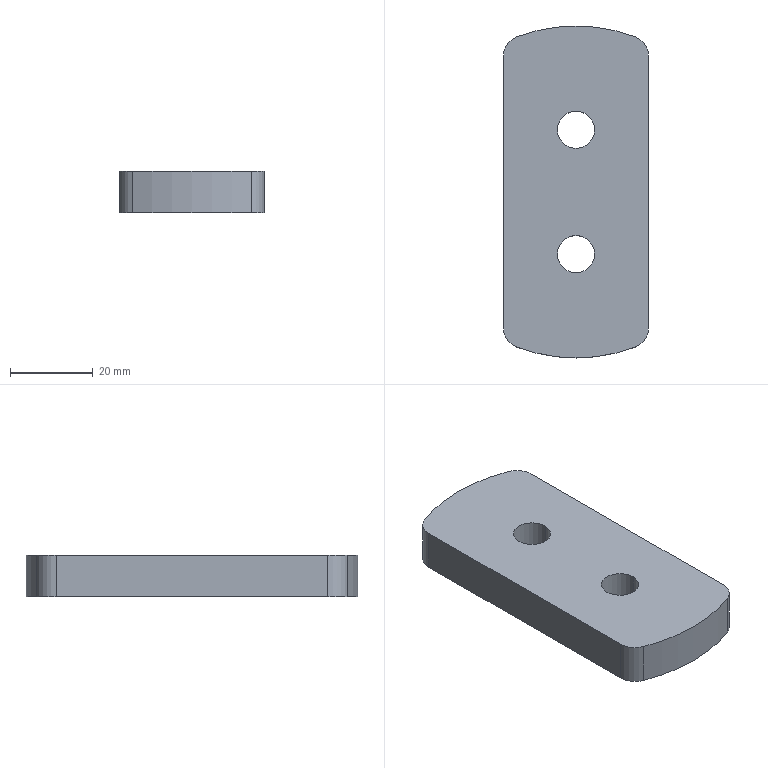Component | SolidWorks | NewTypeCurveBenderReinforcementWheelStopCover-DoubleWheel-1 | 1 solid | 14 faces | box 35 x 80 x 10 mm | volume 25728 mm3 | cylinder 10 | plane 4 | commonest cylinder face diameters 9 x4 10 x4 80 x2
build123d program:
from build123d import *

# Parameters (mm, degrees)
SKETCH1_R           = 4.5
BOSS_EXTRUDE1_DEPTH = 10


with BuildPart() as part:
    # Sketch1 → Boss-Extrude1 (new body)
    with BuildSketch(Plane.XY):
        with BuildLine():
            Line((-17.5, 32.692), (-17.5, -32.692))
            ThreePointArc((-17.5, -32.692), (-16.619, -35.526), (-14.286, -37.362))
            ThreePointArc((-14.286, -37.362), (0, -40), (14.286, -37.362))
            ThreePointArc((14.286, -37.362), (16.619, -35.526), (17.5, -32.692))
            Line((17.5, -32.692), (17.5, 32.692))
            ThreePointArc((17.5, 32.692), (16.619, 35.526), (14.286, 37.362))
            ThreePointArc((14.286, 37.362), (0, 40), (-14.286, 37.362))
            ThreePointArc((-14.286, 37.362), (-16.619, 35.526), (-17.5, 32.692))
        make_face()
        with Locations((0, 15)):
            Circle(SKETCH1_R, mode=Mode.SUBTRACT)
        with Locations(Location((0, -15, 0), (0, 0, 180))):
            Circle(SKETCH1_R, mode=Mode.SUBTRACT)
    extrude(amount=BOSS_EXTRUDE1_DEPTH)


solid = part.part

# Placed as in the assembly
solid = solid.moved(Location((50, -204, 59), (0, 0, 0)))
STEP:
#1=COLOUR_RGB('',0.7922,0.8196,0.9333);
#2=FILL_AREA_STYLE_COLOUR('',#1);
#3=FILL_AREA_STYLE('',(#2));
#4=SURFACE_STYLE_FILL_AREA(#3);
#5=SURFACE_SIDE_STYLE('',(#4));
#6=SURFACE_STYLE_USAGE(.BOTH.,#5);
#7=PRESENTATION_STYLE_ASSIGNMENT((#6));
#8=CARTESIAN_POINT('',(2.146,-8.622,2.323));
#9=VERTEX_POINT('',#8);
#10=CARTESIAN_POINT('',(1.791,-8.622,2.323));
#11=VERTEX_POINT('',#10);
#12=CARTESIAN_POINT('',(1.969,-8.622,2.323));
#13=DIRECTION('',(-0.,0.,-1.));
#14=DIRECTION('',(1.,0.,-0.));
#15=AXIS2_PLACEMENT_3D('',#12,#13,#14);
#16=CIRCLE('',#15,0.1772);
#17=EDGE_CURVE('',#9,#11,#16,.T.);
#18=ORIENTED_EDGE('',*,*,#17,.T.);
#19=CARTESIAN_POINT('',(1.791,-8.622,2.717));
#20=VERTEX_POINT('',#19);
#21=CARTESIAN_POINT('',(1.791,-8.622,2.323));
#22=DIRECTION('',(0.,-0.,1.));
#23=VECTOR('',#22,39.37);
#24=LINE('',#21,#23);
#25=EDGE_CURVE('',#11,#20,#24,.T.);
#26=ORIENTED_EDGE('',*,*,#25,.T.);
#27=CARTESIAN_POINT('',(2.146,-8.622,2.717));
#28=VERTEX_POINT('',#27);
#29=CARTESIAN_POINT('',(1.969,-8.622,2.717));
#30=DIRECTION('',(-0.,0.,-1.));
#31=DIRECTION('',(1.,0.,-0.));
#32=AXIS2_PLACEMENT_3D('',#29,#30,#31);
#33=CIRCLE('',#32,0.1772);
#34=EDGE_CURVE('',#28,#20,#33,.T.);
#35=ORIENTED_EDGE('',*,*,#34,.F.);
#36=CARTESIAN_POINT('',(2.146,-8.622,2.323));
#37=DIRECTION('',(0.,-0.,1.));
#38=VECTOR('',#37,39.37);
#39=LINE('',#36,#38);
#40=EDGE_CURVE('',#9,#28,#39,.T.);
#41=ORIENTED_EDGE('',*,*,#40,.F.);
#42=EDGE_LOOP('',(#18,#26,#35,#41));
#43=FACE_OUTER_BOUND('',#42,.T.);
#44=CARTESIAN_POINT('',(1.969,-8.622,2.323));
#45=DIRECTION('',(0.,-0.,1.));
#46=DIRECTION('',(1.,0.,-0.));
#47=AXIS2_PLACEMENT_3D('',#44,#45,#46);
#48=CYLINDRICAL_SURFACE('',#47,0.1772);
#49=ADVANCED_FACE('',(#43),#48,.F.);
#50=CARTESIAN_POINT('',(2.146,-7.441,2.323));
#51=VERTEX_POINT('',#50);
#52=CARTESIAN_POINT('',(1.791,-7.441,2.323));
#53=VERTEX_POINT('',#52);
#54=CARTESIAN_POINT('',(1.969,-7.441,2.323));
#55=DIRECTION('',(-0.,0.,-1.));
#56=DIRECTION('',(-1.,0.,0.));
#57=AXIS2_PLACEMENT_3D('',#54,#55,#56);
#58=CIRCLE('',#57,0.1772);
#59=EDGE_CURVE('',#51,#53,#58,.T.);
#60=ORIENTED_EDGE('',*,*,#59,.T.);
#61=CARTESIAN_POINT('',(1.791,-7.441,2.717));
#62=VERTEX_POINT('',#61);
#63=CARTESIAN_POINT('',(1.791,-7.441,2.323));
#64=DIRECTION('',(0.,-0.,1.));
#65=VECTOR('',#64,39.37);
#66=LINE('',#63,#65);
#67=EDGE_CURVE('',#53,#62,#66,.T.);
#68=ORIENTED_EDGE('',*,*,#67,.T.);
#69=CARTESIAN_POINT('',(2.146,-7.441,2.717));
#70=VERTEX_POINT('',#69);
#71=CARTESIAN_POINT('',(1.969,-7.441,2.717));
#72=DIRECTION('',(-0.,0.,-1.));
#73=DIRECTION('',(-1.,0.,0.));
#74=AXIS2_PLACEMENT_3D('',#71,#72,#73);
#75=CIRCLE('',#74,0.1772);
#76=EDGE_CURVE('',#70,#62,#75,.T.);
#77=ORIENTED_EDGE('',*,*,#76,.F.);
#78=CARTESIAN_POINT('',(2.146,-7.441,2.323));
#79=DIRECTION('',(0.,-0.,1.));
#80=VECTOR('',#79,39.37);
#81=LINE('',#78,#80);
#82=EDGE_CURVE('',#51,#70,#81,.T.);
#83=ORIENTED_EDGE('',*,*,#82,.F.);
#84=EDGE_LOOP('',(#60,#68,#77,#83));
#85=FACE_OUTER_BOUND('',#84,.T.);
#86=CARTESIAN_POINT('',(1.969,-7.441,2.323));
#87=DIRECTION('',(0.,-0.,1.));
#88=DIRECTION('',(1.,0.,-0.));
#89=AXIS2_PLACEMENT_3D('',#86,#87,#88);
#90=CYLINDRICAL_SURFACE('',#89,0.1772);
#91=ADVANCED_FACE('',(#85),#90,.F.);
#92=CARTESIAN_POINT('',(2.657,-9.319,2.323));
#93=VERTEX_POINT('',#92);
#94=CARTESIAN_POINT('',(2.531,-9.502,2.323));
#95=VERTEX_POINT('',#94);
#96=CARTESIAN_POINT('',(2.461,-9.319,2.323));
#97=DIRECTION('',(-0.,0.,-1.));
#98=DIRECTION('',(1.,0.,-0.));
#99=AXIS2_PLACEMENT_3D('',#96,#97,#98);
#100=CIRCLE('',#99,0.1969);
#101=EDGE_CURVE('',#93,#95,#100,.T.);
#102=ORIENTED_EDGE('',*,*,#101,.T.);
#103=CARTESIAN_POINT('',(1.406,-9.502,2.323));
#104=VERTEX_POINT('',#103);
#105=CARTESIAN_POINT('',(1.969,-8.031,2.323));
#106=DIRECTION('',(-0.,0.,-1.));
#107=DIRECTION('',(-1.,0.,0.));
#108=AXIS2_PLACEMENT_3D('',#105,#106,#107);
#109=CIRCLE('',#108,1.575);
#110=EDGE_CURVE('',#95,#104,#109,.T.);
#111=ORIENTED_EDGE('',*,*,#110,.T.);
#112=CARTESIAN_POINT('',(1.28,-9.319,2.323));
#113=VERTEX_POINT('',#112);
#114=CARTESIAN_POINT('',(1.476,-9.319,2.323));
#115=DIRECTION('',(-0.,0.,-1.));
#116=DIRECTION('',(1.,0.,-0.));
#117=AXIS2_PLACEMENT_3D('',#114,#115,#116);
#118=CIRCLE('',#117,0.1969);
#119=EDGE_CURVE('',#104,#113,#118,.T.);
#120=ORIENTED_EDGE('',*,*,#119,.T.);
#121=CARTESIAN_POINT('',(1.28,-6.744,2.323));
#122=VERTEX_POINT('',#121);
#123=CARTESIAN_POINT('',(1.28,-6.744,2.323));
#124=DIRECTION('',(-0.,1.,0.));
#125=VECTOR('',#124,39.37);
#126=LINE('',#123,#125);
#127=EDGE_CURVE('',#113,#122,#126,.T.);
#128=ORIENTED_EDGE('',*,*,#127,.T.);
#129=CARTESIAN_POINT('',(1.406,-6.561,2.323));
#130=VERTEX_POINT('',#129);
#131=CARTESIAN_POINT('',(1.476,-6.744,2.323));
#132=DIRECTION('',(-0.,0.,-1.));
#133=DIRECTION('',(1.,0.,-0.));
#134=AXIS2_PLACEMENT_3D('',#131,#132,#133);
#135=CIRCLE('',#134,0.1969);
#136=EDGE_CURVE('',#122,#130,#135,.T.);
#137=ORIENTED_EDGE('',*,*,#136,.T.);
#138=CARTESIAN_POINT('',(2.531,-6.561,2.323));
#139=VERTEX_POINT('',#138);
#140=CARTESIAN_POINT('',(1.969,-8.031,2.323));
#141=DIRECTION('',(-0.,0.,-1.));
#142=DIRECTION('',(-1.,0.,0.));
#143=AXIS2_PLACEMENT_3D('',#140,#141,#142);
#144=CIRCLE('',#143,1.575);
#145=EDGE_CURVE('',#130,#139,#144,.T.);
#146=ORIENTED_EDGE('',*,*,#145,.T.);
#147=CARTESIAN_POINT('',(2.657,-6.744,2.323));
#148=VERTEX_POINT('',#147);
#149=CARTESIAN_POINT('',(2.461,-6.744,2.323));
#150=DIRECTION('',(-0.,0.,-1.));
#151=DIRECTION('',(1.,0.,-0.));
#152=AXIS2_PLACEMENT_3D('',#149,#150,#151);
#153=CIRCLE('',#152,0.1969);
#154=EDGE_CURVE('',#139,#148,#153,.T.);
#155=ORIENTED_EDGE('',*,*,#154,.T.);
#156=CARTESIAN_POINT('',(2.657,-6.744,2.323));
#157=DIRECTION('',(-0.,-1.,-0.));
#158=VECTOR('',#157,39.37);
#159=LINE('',#156,#158);
#160=EDGE_CURVE('',#148,#93,#159,.T.);
#161=ORIENTED_EDGE('',*,*,#160,.T.);
#162=EDGE_LOOP('',(#102,#111,#120,#128,#137,#146,#155,#161));
#163=FACE_OUTER_BOUND('',#162,.T.);
#164=ORIENTED_EDGE('',*,*,#59,.F.);
#165=CARTESIAN_POINT('',(1.969,-7.441,2.323));
#166=DIRECTION('',(-0.,0.,-1.));
#167=DIRECTION('',(-1.,0.,0.));
#168=AXIS2_PLACEMENT_3D('',#165,#166,#167);
#169=CIRCLE('',#168,0.1772);
#170=EDGE_CURVE('',#53,#51,#169,.T.);
#171=ORIENTED_EDGE('',*,*,#170,.F.);
#172=EDGE_LOOP('',(#164,#171));
#173=FACE_BOUND('',#172,.T.);
#174=ORIENTED_EDGE('',*,*,#17,.F.);
#175=CARTESIAN_POINT('',(1.969,-8.622,2.323));
#176=DIRECTION('',(-0.,0.,-1.));
#177=DIRECTION('',(1.,0.,-0.));
#178=AXIS2_PLACEMENT_3D('',#175,#176,#177);
#179=CIRCLE('',#178,0.1772);
#180=EDGE_CURVE('',#11,#9,#179,.T.);
#181=ORIENTED_EDGE('',*,*,#180,.F.);
#182=EDGE_LOOP('',(#174,#181));
#183=FACE_BOUND('',#182,.T.);
#184=CARTESIAN_POINT('',(2.461,-9.319,2.323));
#185=DIRECTION('',(0.,-0.,1.));
#186=DIRECTION('',(1.,-0.,-0.));
#187=AXIS2_PLACEMENT_3D('',#184,#185,#186);
#188=PLANE('',#187);
#189=ADVANCED_FACE('',(#163,#173,#183),#188,.F.);
#190=ORIENTED_EDGE('',*,*,#76,.T.);
#191=CARTESIAN_POINT('',(1.969,-7.441,2.717));
#192=DIRECTION('',(-0.,0.,-1.));
#193=DIRECTION('',(-1.,0.,0.));
#194=AXIS2_PLACEMENT_3D('',#191,#192,#193);
#195=CIRCLE('',#194,0.1772);
#196=EDGE_CURVE('',#62,#70,#195,.T.);
#197=ORIENTED_EDGE('',*,*,#196,.T.);
#198=EDGE_LOOP('',(#190,#197));
#199=FACE_BOUND('',#198,.T.);
#200=CARTESIAN_POINT('',(2.657,-9.319,2.717));
#201=VERTEX_POINT('',#200);
#202=CARTESIAN_POINT('',(2.531,-9.502,2.717));
#203=VERTEX_POINT('',#202);
#204=CARTESIAN_POINT('',(2.461,-9.319,2.717));
#205=DIRECTION('',(-0.,0.,-1.));
#206=DIRECTION('',(1.,0.,-0.));
#207=AXIS2_PLACEMENT_3D('',#204,#205,#206);
#208=CIRCLE('',#207,0.1969);
#209=EDGE_CURVE('',#201,#203,#208,.T.);
#210=ORIENTED_EDGE('',*,*,#209,.F.);
#211=CARTESIAN_POINT('',(2.657,-6.744,2.717));
#212=VERTEX_POINT('',#211);
#213=CARTESIAN_POINT('',(2.657,-6.744,2.717));
#214=DIRECTION('',(-0.,-1.,-0.));
#215=VECTOR('',#214,39.37);
#216=LINE('',#213,#215);
#217=EDGE_CURVE('',#212,#201,#216,.T.);
#218=ORIENTED_EDGE('',*,*,#217,.F.);
#219=CARTESIAN_POINT('',(2.531,-6.561,2.717));
#220=VERTEX_POINT('',#219);
#221=CARTESIAN_POINT('',(2.461,-6.744,2.717));
#222=DIRECTION('',(-0.,0.,-1.));
#223=DIRECTION('',(1.,0.,-0.));
#224=AXIS2_PLACEMENT_3D('',#221,#222,#223);
#225=CIRCLE('',#224,0.1969);
#226=EDGE_CURVE('',#220,#212,#225,.T.);
#227=ORIENTED_EDGE('',*,*,#226,.F.);
#228=CARTESIAN_POINT('',(1.406,-6.561,2.717));
#229=VERTEX_POINT('',#228);
#230=CARTESIAN_POINT('',(1.969,-8.031,2.717));
#231=DIRECTION('',(-0.,0.,-1.));
#232=DIRECTION('',(-1.,0.,0.));
#233=AXIS2_PLACEMENT_3D('',#230,#231,#232);
#234=CIRCLE('',#233,1.575);
#235=EDGE_CURVE('',#229,#220,#234,.T.);
#236=ORIENTED_EDGE('',*,*,#235,.F.);
#237=CARTESIAN_POINT('',(1.28,-6.744,2.717));
#238=VERTEX_POINT('',#237);
#239=CARTESIAN_POINT('',(1.476,-6.744,2.717));
#240=DIRECTION('',(-0.,0.,-1.));
#241=DIRECTION('',(1.,0.,-0.));
#242=AXIS2_PLACEMENT_3D('',#239,#240,#241);
#243=CIRCLE('',#242,0.1969);
#244=EDGE_CURVE('',#238,#229,#243,.T.);
#245=ORIENTED_EDGE('',*,*,#244,.F.);
#246=CARTESIAN_POINT('',(1.28,-9.319,2.717));
#247=VERTEX_POINT('',#246);
#248=CARTESIAN_POINT('',(1.28,-6.744,2.717));
#249=DIRECTION('',(-0.,1.,0.));
#250=VECTOR('',#249,39.37);
#251=LINE('',#248,#250);
#252=EDGE_CURVE('',#247,#238,#251,.T.);
#253=ORIENTED_EDGE('',*,*,#252,.F.);
#254=CARTESIAN_POINT('',(1.406,-9.502,2.717));
#255=VERTEX_POINT('',#254);
#256=CARTESIAN_POINT('',(1.476,-9.319,2.717));
#257=DIRECTION('',(-0.,0.,-1.));
#258=DIRECTION('',(1.,0.,-0.));
#259=AXIS2_PLACEMENT_3D('',#256,#257,#258);
#260=CIRCLE('',#259,0.1969);
#261=EDGE_CURVE('',#255,#247,#260,.T.);
#262=ORIENTED_EDGE('',*,*,#261,.F.);
#263=CARTESIAN_POINT('',(1.969,-8.031,2.717));
#264=DIRECTION('',(-0.,0.,-1.));
#265=DIRECTION('',(-1.,0.,0.));
#266=AXIS2_PLACEMENT_3D('',#263,#264,#265);
#267=CIRCLE('',#266,1.575);
#268=EDGE_CURVE('',#203,#255,#267,.T.);
#269=ORIENTED_EDGE('',*,*,#268,.F.);
#270=EDGE_LOOP('',(#210,#218,#227,#236,#245,#253,#262,#269));
#271=FACE_OUTER_BOUND('',#270,.T.);
#272=ORIENTED_EDGE('',*,*,#34,.T.);
#273=CARTESIAN_POINT('',(1.969,-8.622,2.717));
#274=DIRECTION('',(-0.,0.,-1.));
#275=DIRECTION('',(1.,0.,-0.));
#276=AXIS2_PLACEMENT_3D('',#273,#274,#275);
#277=CIRCLE('',#276,0.1772);
#278=EDGE_CURVE('',#20,#28,#277,.T.);
#279=ORIENTED_EDGE('',*,*,#278,.T.);
#280=EDGE_LOOP('',(#272,#279));
#281=FACE_BOUND('',#280,.T.);
#282=CARTESIAN_POINT('',(2.461,-9.319,2.717));
#283=DIRECTION('',(0.,-0.,1.));
#284=DIRECTION('',(1.,-0.,-0.));
#285=AXIS2_PLACEMENT_3D('',#282,#283,#284);
#286=PLANE('',#285);
#287=ADVANCED_FACE('',(#199,#271,#281),#286,.T.);
#288=ORIENTED_EDGE('',*,*,#209,.T.);
#289=CARTESIAN_POINT('',(2.531,-9.502,2.323));
#290=DIRECTION('',(0.,-0.,1.));
#291=VECTOR('',#290,39.37);
#292=LINE('',#289,#291);
#293=EDGE_CURVE('',#95,#203,#292,.T.);
#294=ORIENTED_EDGE('',*,*,#293,.F.);
#295=ORIENTED_EDGE('',*,*,#101,.F.);
#296=CARTESIAN_POINT('',(2.657,-9.319,2.323));
#297=DIRECTION('',(0.,-0.,1.));
#298=VECTOR('',#297,39.37);
#299=LINE('',#296,#298);
#300=EDGE_CURVE('',#93,#201,#299,.T.);
#301=ORIENTED_EDGE('',*,*,#300,.T.);
#302=EDGE_LOOP('',(#288,#294,#295,#301));
#303=FACE_OUTER_BOUND('',#302,.T.);
#304=CARTESIAN_POINT('',(2.461,-9.319,2.323));
#305=DIRECTION('',(0.,-0.,1.));
#306=DIRECTION('',(1.,0.,-0.));
#307=AXIS2_PLACEMENT_3D('',#304,#305,#306);
#308=CYLINDRICAL_SURFACE('',#307,0.1969);
#309=ADVANCED_FACE('',(#303),#308,.T.);
#310=ORIENTED_EDGE('',*,*,#268,.T.);
#311=CARTESIAN_POINT('',(1.406,-9.502,2.323));
#312=DIRECTION('',(0.,-0.,1.));
#313=VECTOR('',#312,39.37);
#314=LINE('',#311,#313);
#315=EDGE_CURVE('',#104,#255,#314,.T.);
#316=ORIENTED_EDGE('',*,*,#315,.F.);
#317=ORIENTED_EDGE('',*,*,#110,.F.);
#318=ORIENTED_EDGE('',*,*,#293,.T.);
#319=EDGE_LOOP('',(#310,#316,#317,#318));
#320=FACE_OUTER_BOUND('',#319,.T.);
#321=CARTESIAN_POINT('',(1.969,-8.031,2.323));
#322=DIRECTION('',(0.,-0.,1.));
#323=DIRECTION('',(1.,0.,-0.));
#324=AXIS2_PLACEMENT_3D('',#321,#322,#323);
#325=CYLINDRICAL_SURFACE('',#324,1.575);
#326=ADVANCED_FACE('',(#320),#325,.T.);
#327=ORIENTED_EDGE('',*,*,#261,.T.);
#328=CARTESIAN_POINT('',(1.28,-9.319,2.323));
#329=DIRECTION('',(0.,-0.,1.));
#330=VECTOR('',#329,39.37);
#331=LINE('',#328,#330);
#332=EDGE_CURVE('',#113,#247,#331,.T.);
#333=ORIENTED_EDGE('',*,*,#332,.F.);
#334=ORIENTED_EDGE('',*,*,#119,.F.);
#335=ORIENTED_EDGE('',*,*,#315,.T.);
#336=EDGE_LOOP('',(#327,#333,#334,#335));
#337=FACE_OUTER_BOUND('',#336,.T.);
#338=CARTESIAN_POINT('',(1.476,-9.319,2.323));
#339=DIRECTION('',(0.,-0.,1.));
#340=DIRECTION('',(1.,0.,-0.));
#341=AXIS2_PLACEMENT_3D('',#338,#339,#340);
#342=CYLINDRICAL_SURFACE('',#341,0.1969);
#343=ADVANCED_FACE('',(#337),#342,.T.);
#344=ORIENTED_EDGE('',*,*,#252,.T.);
#345=CARTESIAN_POINT('',(1.28,-6.744,2.323));
#346=DIRECTION('',(0.,-0.,1.));
#347=VECTOR('',#346,39.37);
#348=LINE('',#345,#347);
#349=EDGE_CURVE('',#122,#238,#348,.T.);
#350=ORIENTED_EDGE('',*,*,#349,.F.);
#351=ORIENTED_EDGE('',*,*,#127,.F.);
#352=ORIENTED_EDGE('',*,*,#332,.T.);
#353=EDGE_LOOP('',(#344,#350,#351,#352));
#354=FACE_OUTER_BOUND('',#353,.T.);
#355=CARTESIAN_POINT('',(1.28,-6.744,2.323));
#356=DIRECTION('',(1.,0.,-0.));
#357=DIRECTION('',(0.,-1.,-0.));
#358=AXIS2_PLACEMENT_3D('',#355,#356,#357);
#359=PLANE('',#358);
#360=ADVANCED_FACE('',(#354),#359,.F.);
#361=ORIENTED_EDGE('',*,*,#244,.T.);
#362=CARTESIAN_POINT('',(1.406,-6.561,2.323));
#363=DIRECTION('',(0.,-0.,1.));
#364=VECTOR('',#363,39.37);
#365=LINE('',#362,#364);
#366=EDGE_CURVE('',#130,#229,#365,.T.);
#367=ORIENTED_EDGE('',*,*,#366,.F.);
#368=ORIENTED_EDGE('',*,*,#136,.F.);
#369=ORIENTED_EDGE('',*,*,#349,.T.);
#370=EDGE_LOOP('',(#361,#367,#368,#369));
#371=FACE_OUTER_BOUND('',#370,.T.);
#372=CARTESIAN_POINT('',(1.476,-6.744,2.323));
#373=DIRECTION('',(0.,-0.,1.));
#374=DIRECTION('',(1.,0.,-0.));
#375=AXIS2_PLACEMENT_3D('',#372,#373,#374);
#376=CYLINDRICAL_SURFACE('',#375,0.1969);
#377=ADVANCED_FACE('',(#371),#376,.T.);
#378=ORIENTED_EDGE('',*,*,#235,.T.);
#379=CARTESIAN_POINT('',(2.531,-6.561,2.323));
#380=DIRECTION('',(0.,-0.,1.));
#381=VECTOR('',#380,39.37);
#382=LINE('',#379,#381);
#383=EDGE_CURVE('',#139,#220,#382,.T.);
#384=ORIENTED_EDGE('',*,*,#383,.F.);
#385=ORIENTED_EDGE('',*,*,#145,.F.);
#386=ORIENTED_EDGE('',*,*,#366,.T.);
#387=EDGE_LOOP('',(#378,#384,#385,#386));
#388=FACE_OUTER_BOUND('',#387,.T.);
#389=CARTESIAN_POINT('',(1.969,-8.031,2.323));
#390=DIRECTION('',(0.,-0.,1.));
#391=DIRECTION('',(1.,0.,-0.));
#392=AXIS2_PLACEMENT_3D('',#389,#390,#391);
#393=CYLINDRICAL_SURFACE('',#392,1.575);
#394=ADVANCED_FACE('',(#388),#393,.T.);
#395=ORIENTED_EDGE('',*,*,#226,.T.);
#396=CARTESIAN_POINT('',(2.657,-6.744,2.323));
#397=DIRECTION('',(0.,-0.,1.));
#398=VECTOR('',#397,39.37);
#399=LINE('',#396,#398);
#400=EDGE_CURVE('',#148,#212,#399,.T.);
#401=ORIENTED_EDGE('',*,*,#400,.F.);
#402=ORIENTED_EDGE('',*,*,#154,.F.);
#403=ORIENTED_EDGE('',*,*,#383,.T.);
#404=EDGE_LOOP('',(#395,#401,#402,#403));
#405=FACE_OUTER_BOUND('',#404,.T.);
#406=CARTESIAN_POINT('',(2.461,-6.744,2.323));
#407=DIRECTION('',(0.,-0.,1.));
#408=DIRECTION('',(1.,0.,-0.));
#409=AXIS2_PLACEMENT_3D('',#406,#407,#408);
#410=CYLINDRICAL_SURFACE('',#409,0.1969);
#411=ADVANCED_FACE('',(#405),#410,.T.);
#412=ORIENTED_EDGE('',*,*,#217,.T.);
#413=ORIENTED_EDGE('',*,*,#300,.F.);
#414=ORIENTED_EDGE('',*,*,#160,.F.);
#415=ORIENTED_EDGE('',*,*,#400,.T.);
#416=EDGE_LOOP('',(#412,#413,#414,#415));
#417=FACE_OUTER_BOUND('',#416,.T.);
#418=CARTESIAN_POINT('',(2.657,-6.744,2.323));
#419=DIRECTION('',(-1.,0.,0.));
#420=DIRECTION('',(0.,1.,0.));
#421=AXIS2_PLACEMENT_3D('',#418,#419,#420);
#422=PLANE('',#421);
#423=ADVANCED_FACE('',(#417),#422,.F.);
#424=ORIENTED_EDGE('',*,*,#67,.F.);
#425=ORIENTED_EDGE('',*,*,#170,.T.);
#426=ORIENTED_EDGE('',*,*,#82,.T.);
#427=ORIENTED_EDGE('',*,*,#196,.F.);
#428=EDGE_LOOP('',(#424,#425,#426,#427));
#429=FACE_OUTER_BOUND('',#428,.T.);
#430=CARTESIAN_POINT('',(1.969,-7.441,2.323));
#431=DIRECTION('',(0.,-0.,1.));
#432=DIRECTION('',(1.,0.,-0.));
#433=AXIS2_PLACEMENT_3D('',#430,#431,#432);
#434=CYLINDRICAL_SURFACE('',#433,0.1772);
#435=ADVANCED_FACE('',(#429),#434,.F.);
#436=ORIENTED_EDGE('',*,*,#25,.F.);
#437=ORIENTED_EDGE('',*,*,#180,.T.);
#438=ORIENTED_EDGE('',*,*,#40,.T.);
#439=ORIENTED_EDGE('',*,*,#278,.F.);
#440=EDGE_LOOP('',(#436,#437,#438,#439));
#441=FACE_OUTER_BOUND('',#440,.T.);
#442=CARTESIAN_POINT('',(1.969,-8.622,2.323));
#443=DIRECTION('',(0.,-0.,1.));
#444=DIRECTION('',(1.,0.,-0.));
#445=AXIS2_PLACEMENT_3D('',#442,#443,#444);
#446=CYLINDRICAL_SURFACE('',#445,0.1772);
#447=ADVANCED_FACE('',(#441),#446,.F.);
#448=CLOSED_SHELL('',(#49,#91,#189,#287,#309,#326,#343,#360,#377,#394,#411,#423,#435,#447));
#449=MANIFOLD_SOLID_BREP('',#448);
#450=STYLED_ITEM('',(#7),#449);
#451=(LENGTH_UNIT()NAMED_UNIT(*)SI_UNIT($,.METRE.));
#452=LENGTH_MEASURE_WITH_UNIT(LENGTH_MEASURE(0.0254),#451);
#453=DIMENSIONAL_EXPONENTS(1.,0.,0.,0.,0.,0.,0.);
#454=(CONVERSION_BASED_UNIT('',#452)LENGTH_UNIT()NAMED_UNIT(#453));
#455=UNCERTAINTY_MEASURE_WITH_UNIT(LENGTH_MEASURE(0.00001),#454,'','');
#456=(NAMED_UNIT(*)PLANE_ANGLE_UNIT()SI_UNIT($,.RADIAN.));
#457=(NAMED_UNIT(*)SI_UNIT($,.STERADIAN.)SOLID_ANGLE_UNIT());
#458=(GEOMETRIC_REPRESENTATION_CONTEXT(3)GLOBAL_UNCERTAINTY_ASSIGNED_CONTEXT((#455))GLOBAL_UNIT_ASSIGNED_CONTEXT((#454,#456,#457))REPRESENTATION_CONTEXT('',''));
#459=MECHANICAL_DESIGN_GEOMETRIC_PRESENTATION_REPRESENTATION('',(#450),#458);
#460=PRESENTATION_LAYER_ASSIGNMENT('','',(#450));
#461=CARTESIAN_POINT('',(0.,0.,0.));
#462=DIRECTION('',(0.,0.,1.));
#463=DIRECTION('',(1.,0.,0.));
#464=AXIS2_PLACEMENT_3D('',#461,#462,#463);
#465=(LENGTH_UNIT()NAMED_UNIT(*)SI_UNIT($,.METRE.));
#466=LENGTH_MEASURE_WITH_UNIT(LENGTH_MEASURE(0.0254),#465);
#467=DIMENSIONAL_EXPONENTS(1.,0.,0.,0.,0.,0.,0.);
#468=(CONVERSION_BASED_UNIT('',#466)LENGTH_UNIT()NAMED_UNIT(#467));
#469=UNCERTAINTY_MEASURE_WITH_UNIT(LENGTH_MEASURE(0.00001),#468,'','');
#470=(NAMED_UNIT(*)PLANE_ANGLE_UNIT()SI_UNIT($,.RADIAN.));
#471=(NAMED_UNIT(*)SI_UNIT($,.STERADIAN.)SOLID_ANGLE_UNIT());
#472=(GEOMETRIC_REPRESENTATION_CONTEXT(3)GLOBAL_UNCERTAINTY_ASSIGNED_CONTEXT((#469))GLOBAL_UNIT_ASSIGNED_CONTEXT((#468,#470,#471))REPRESENTATION_CONTEXT('',''));
#473=ADVANCED_BREP_SHAPE_REPRESENTATION('',(#449,#464),#472);